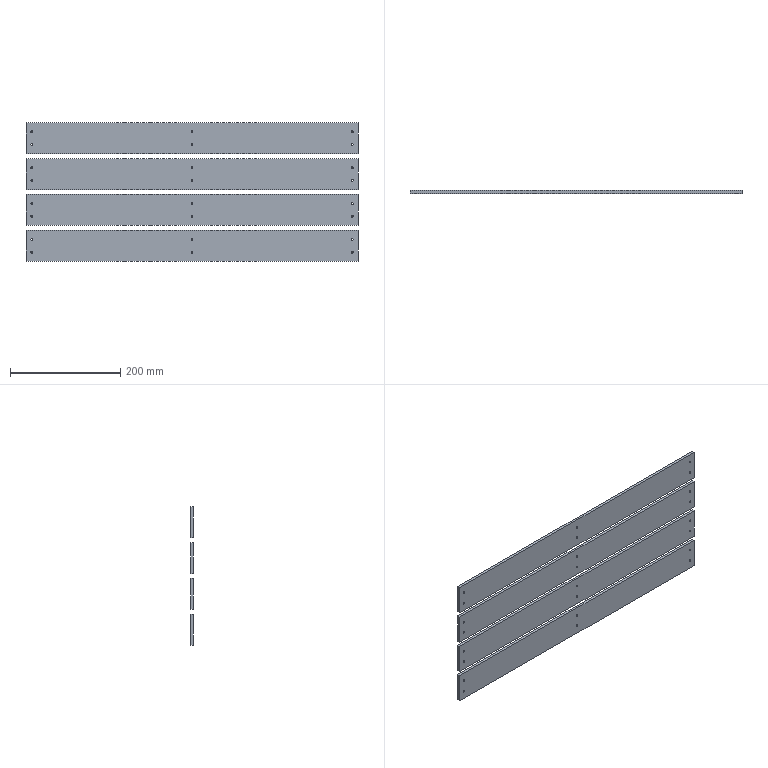CAM job | Mastercam | mm | 4 operations | part box 601 x 5 x 251
1. Contour (Ramp) | 3 - 3 平铣刀
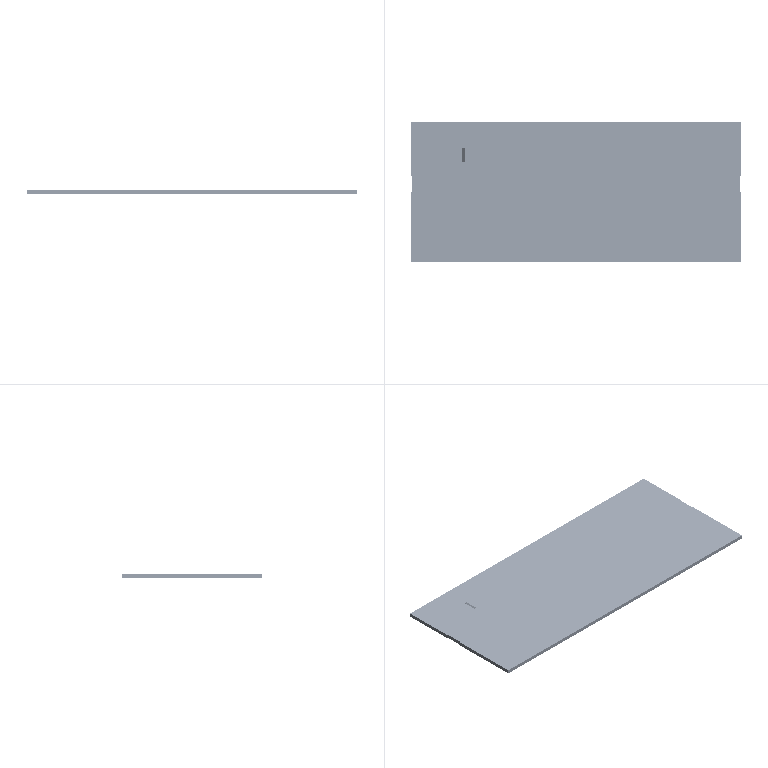2. Contour (2D) | 3 - 3 平铣刀
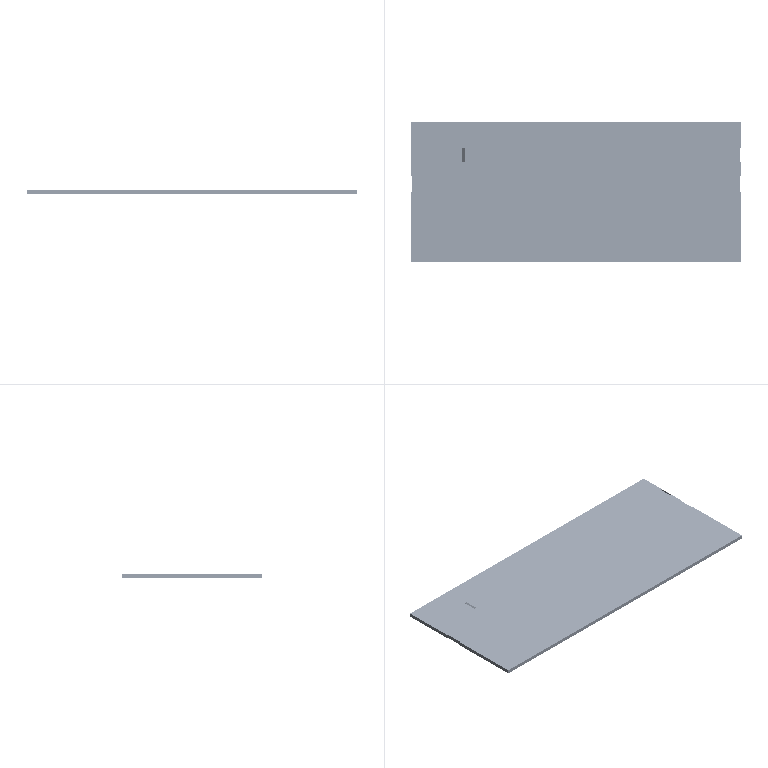3. Drill/Counterbore | 7 - 4 倒角刀
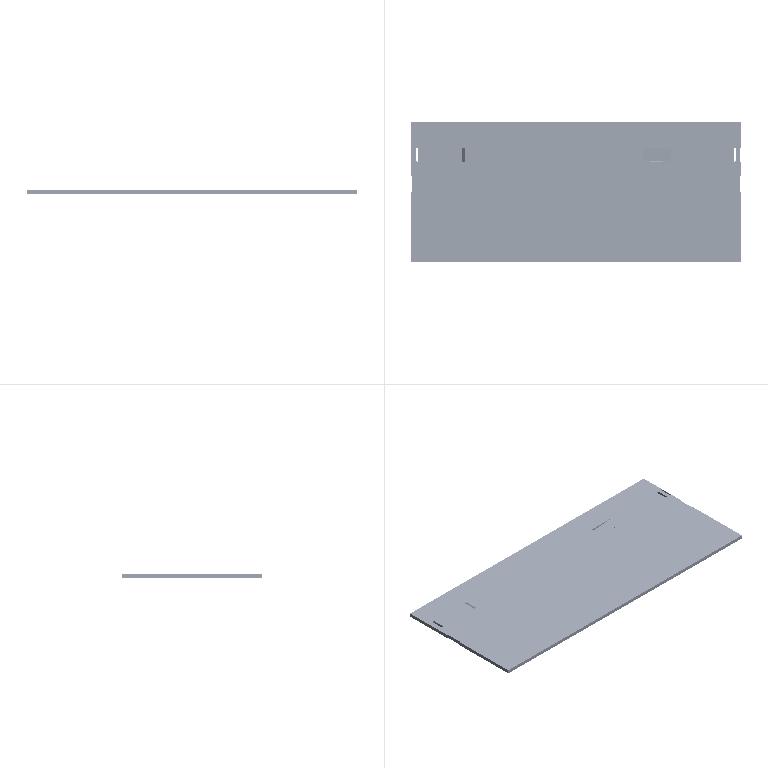4. Contour (2D chamfer) | 7 - 4 倒角刀